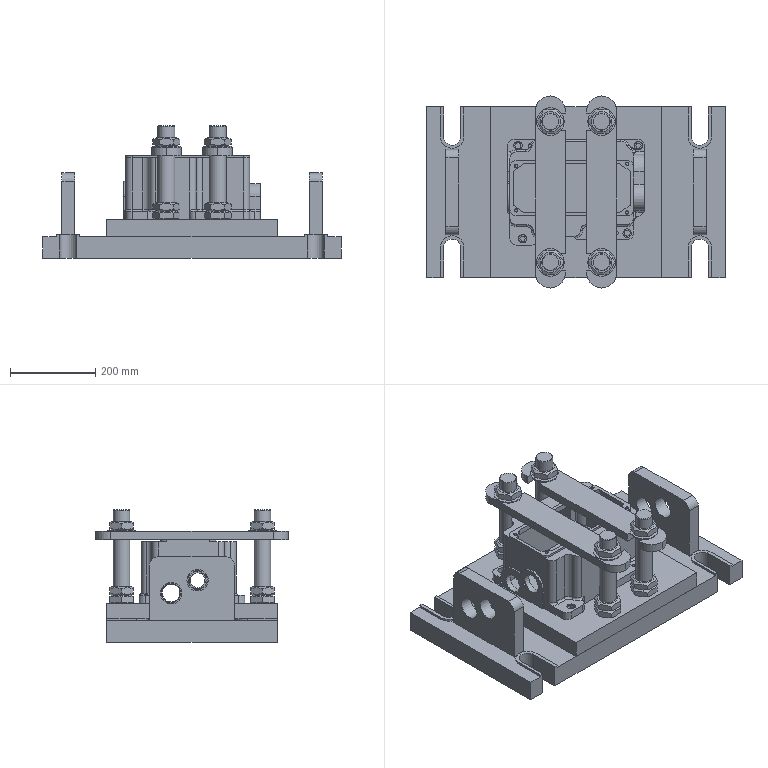Assembly | NX | mm | 33 component files | 33 solids | 609 faces | box 700 x 450 x 310 mm | volume 25568767 mm3 | plane 314 | cylinder 212 | cone 70 | torus 11 | spline 2 | commonest cylinder face diameters 40 x37 2 x36 30 x30 14 x19 10 x14 70 x10 6.8 x9 13.998 x6
Bill of materials:
unnamed part 1 | 1 |  | Flat square plate of uniform thickness with four larger round holes and two smaller round holes.
unnamed part 2 | 12 |  | Thin hexagonal ring with a large central round bore and chamfered corners on both faces, similar in form to a thin hex nut.
unnamed part 3 | 1 |  | Open-top rectangular box housing with a stepped top rim, a flanged base with mounting holes, an internal wall, and a raised side boss with two round openings.
unnamed part 4 | 1 |  | Rectangular plate with four open-ended U-slots at the short ends, stepped areas around the slots, and a pattern of larger and smaller round holes.
unnamed part 5 | 2 |  | Headed cylindrical fastener shape: a short cylindrical head with a hexagonal socket recess on a long plain shank with a chamfered end, similar in form to a socket head cap screw.
unnamed part 6 | 1 |  | Thick rectangular block or plate with two adjacent rounded corners and two round through holes offset diagonally from each other.
unnamed part 7 | 4 |  | Plain solid cylindrical rod or pin with flat ends, possibly with very small edge breaks.
unnamed part 8 | 2 |  | Long flat bar with fully rounded ends and an open U-slot near each end, both slots opening to the same long edge.
unnamed part 9 | 4 |  | Thick rectangular block or plate with two adjacent rounded corners and two round through holes offset diagonally from each other.
unnamed part 10 | 1 |  | Thin flat annular ring with a large central hole, similar in form to a plain flat washer or shim.
unnamed part 11 | 4 |  | Headed pin: a short, wide cylindrical head with a smaller cylindrical shaft that has a chamfered free end; no drive recess is visible.
Mates:
1. fix | fixture_base 1 component
2. touch align | locating_base_plate 1 face | fixture_base 1 face
3. center | locating_base_plate 1 face | locating_base_plate 1 face | fixture_base 1 face | fixture_base 1 face
4. center | locating_base_plate 1 face | locating_base_plate 1 face | fixture_base 1 face | fixture_base 1 face
5. touch align | locating_base_plate 1 face | lathe_feed_box 1 face
6. center | lathe_feed_box 1 face | lathe_feed_box 1 face | locating_base_plate 1 face | locating_base_plate 1 face
7. center | lathe_feed_box 1 face | lathe_feed_box 1 face | locating_base_plate 1 face | locating_base_plate 1 face
8. concentric | screw_M14 2 edge | lathe_feed_box 1 edge
9. concentric | screw_M14 1 edge | lathe_feed_box 1 edge
10. parallel | screw_M14 1 face | lathe_feed_box 1 face
11. parallel | screw_M14 2 face | locating_base_plate 1 face
12. concentric | stud 4 edge | fixture_base 1 edge
13. concentric | stud 3 edge | fixture_base 1 edge
14. concentric | stud 2 edge | fixture_base 1 edge
15. concentric | stud 1 edge | fixture_base 1 edge
16. concentric | washer 4 arc | stud 1 arc
17. concentric | washer 3 arc | stud 3 arc
18. concentric | washer 2 arc | stud 4 arc
19. concentric | nut 12 edge | washer 3 edge
20. concentric | washer 2 edge | nut 11 edge
21. concentric | nut 10 edge | washer 4 edge
22. concentric | locating_base_plate 1 edge | nut 9 edge
23. parallel | nut 9 face | locating_base_plate 1 face
24. concentric | nut 9 edge | nut 8 edge
25. parallel | nut 8 face | locating_base_plate 1 face
26. concentric | locating_base_plate 1 edge | nut 7 edge
27. concentric | nut 7 edge | nut 6 edge
28. parallel | nut 6 face | locating_base_plate 1 face
29. concentric | locating_base_plate 1 edge | nut 5 edge
30. parallel | nut 5 face | locating_base_plate 1 face
31. concentric | nut 5 edge | nut 4 edge
32. parallel | nut 4 face | locating_base_plate 1 face
33. concentric | locating_base_plate 1 edge | nut 3 edge
34. concentric | nut 3 edge | nut 2 edge
35. parallel | nut 2 face | locating_base_plate 1 face
36. center | template 1 face | template 1 face | fixture_base 1 face | fixture_base 1 face
37. touch align | fixture_base 1 face | template 1 face
38. center | template 1 face | template 1 face | fixture_base 1 face | fixture_base 1 face
39. parallel | template_2 1 face | fixture_base 1 face
40. center | template_2 1 face | template_2 1 face | fixture_base 1 face | fixture_base 1 face
41. touch align | fixture_base 1 face | template_2 1 face
42. concentric | template_locating_screw 4 edge | fixture_base 1 edge
43. concentric | template_locating_screw 3 edge | fixture_base 1 edge
44. concentric | template_locating_screw 2 edge | fixture_base 1 edge
45. concentric | template_locating_screw 1 edge | fixture_base 1 edge
46. center | template_2 1 face | template_2 1 face | template 1 face | template 1 face
47. concentric | clamp_plate 2 arc | washer 2 edge
48. parallel | clamp_plate 2 face | template 1 face
49. concentric | clamp_plate 1 arc | washer 3 edge
50. parallel | clamp_plate 1 face | lathe_feed_box 1 face
51. concentric | washer 1 arc | clamp_plate 1 edge
52. concentric | washer 1 edge | nut 1 edge